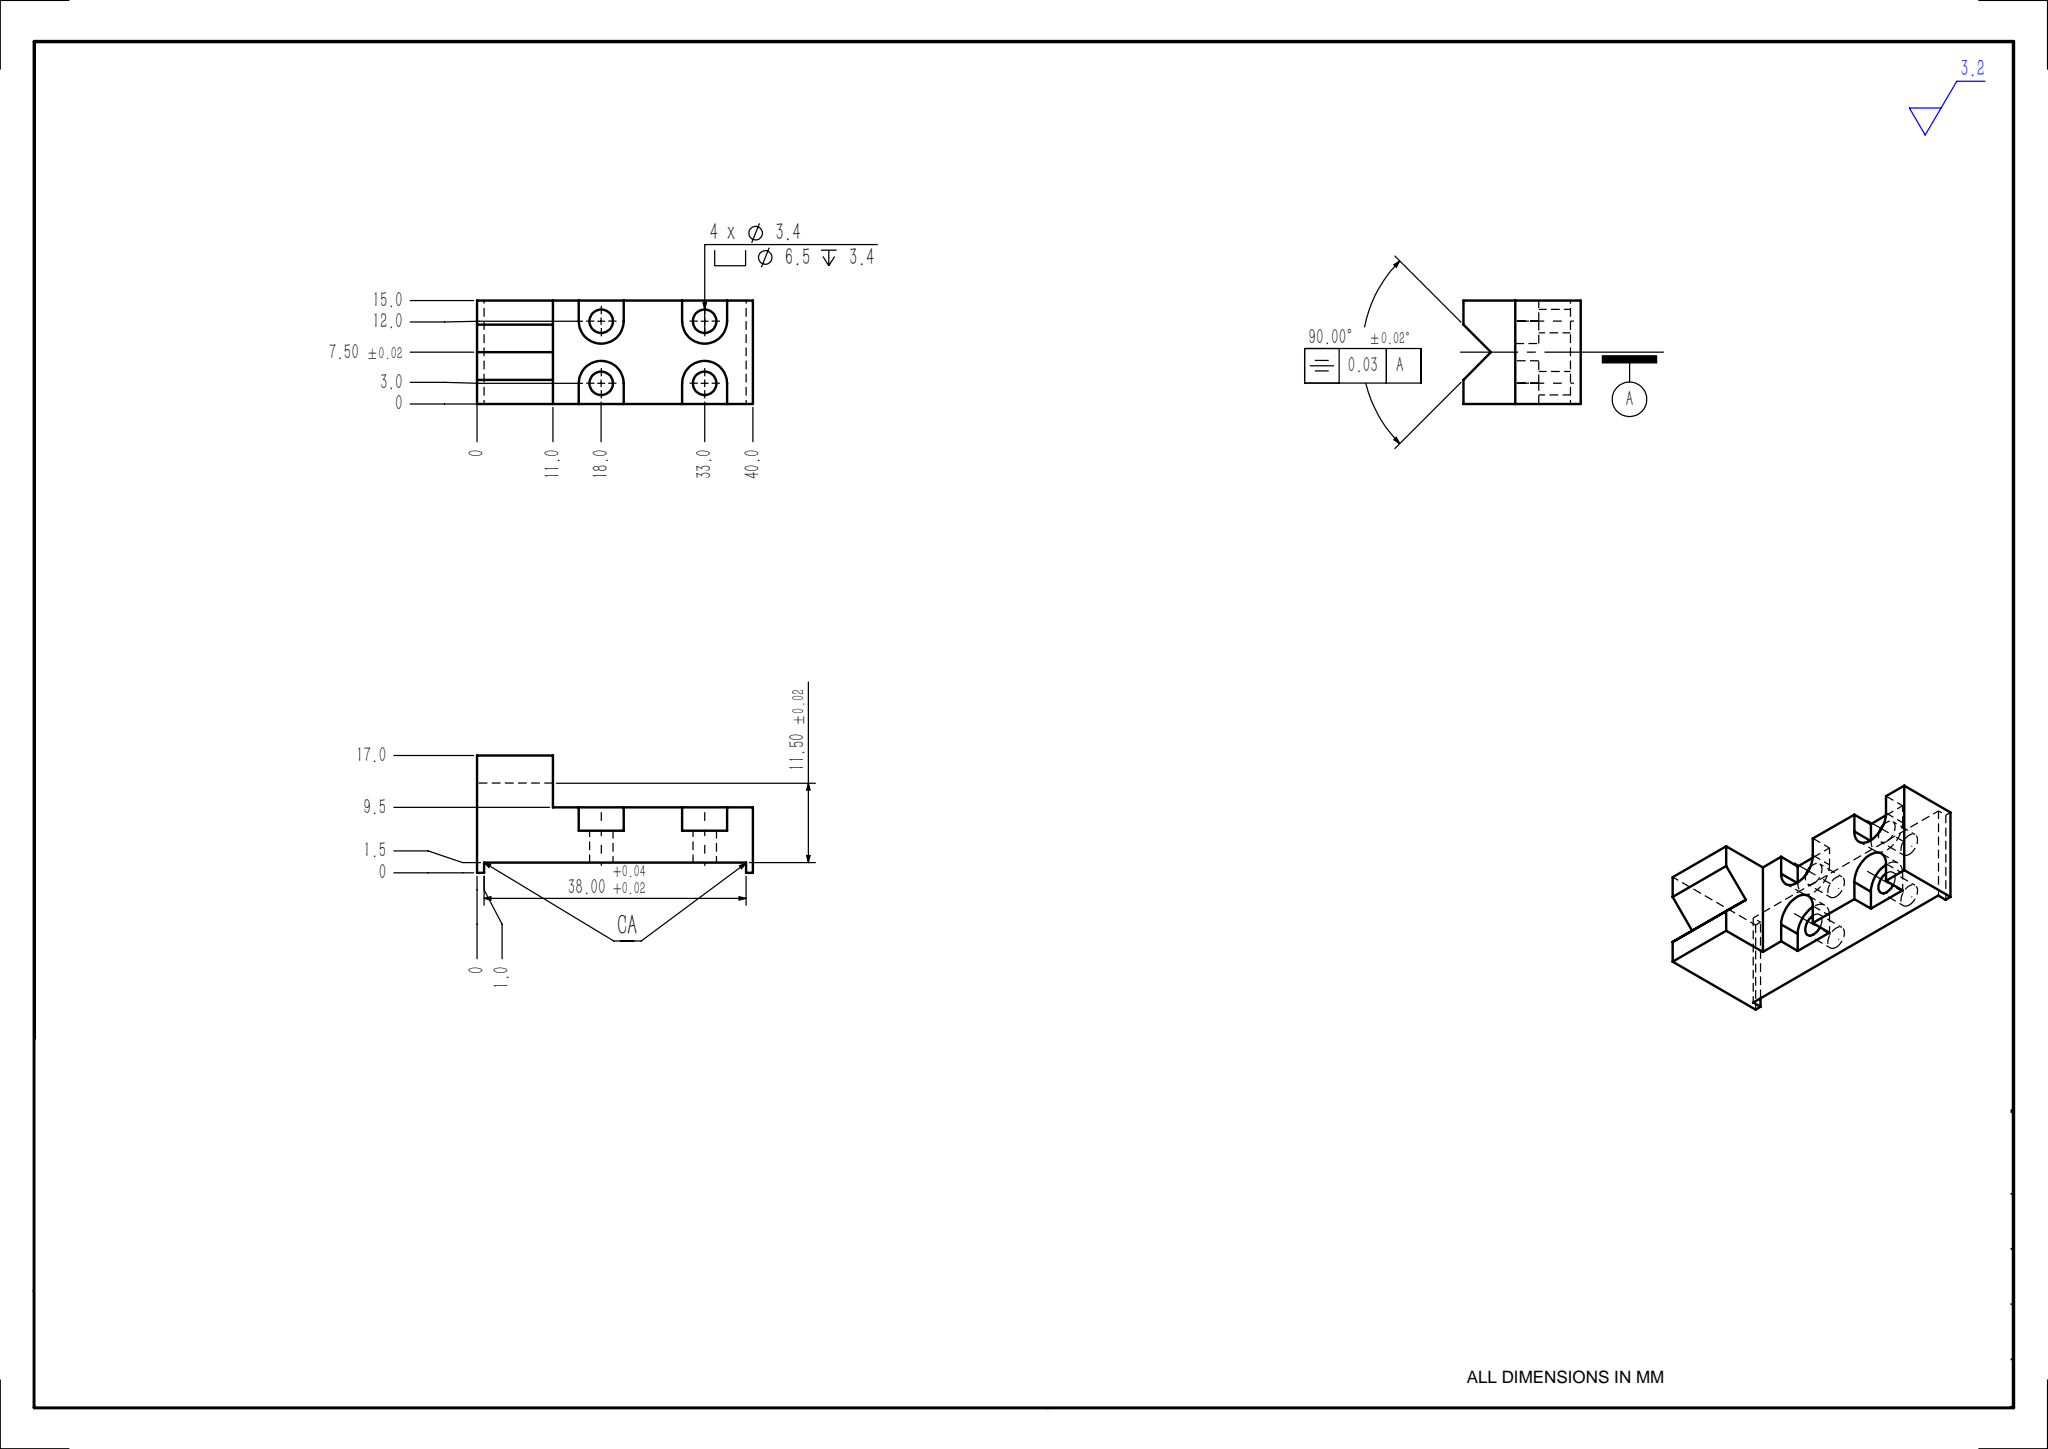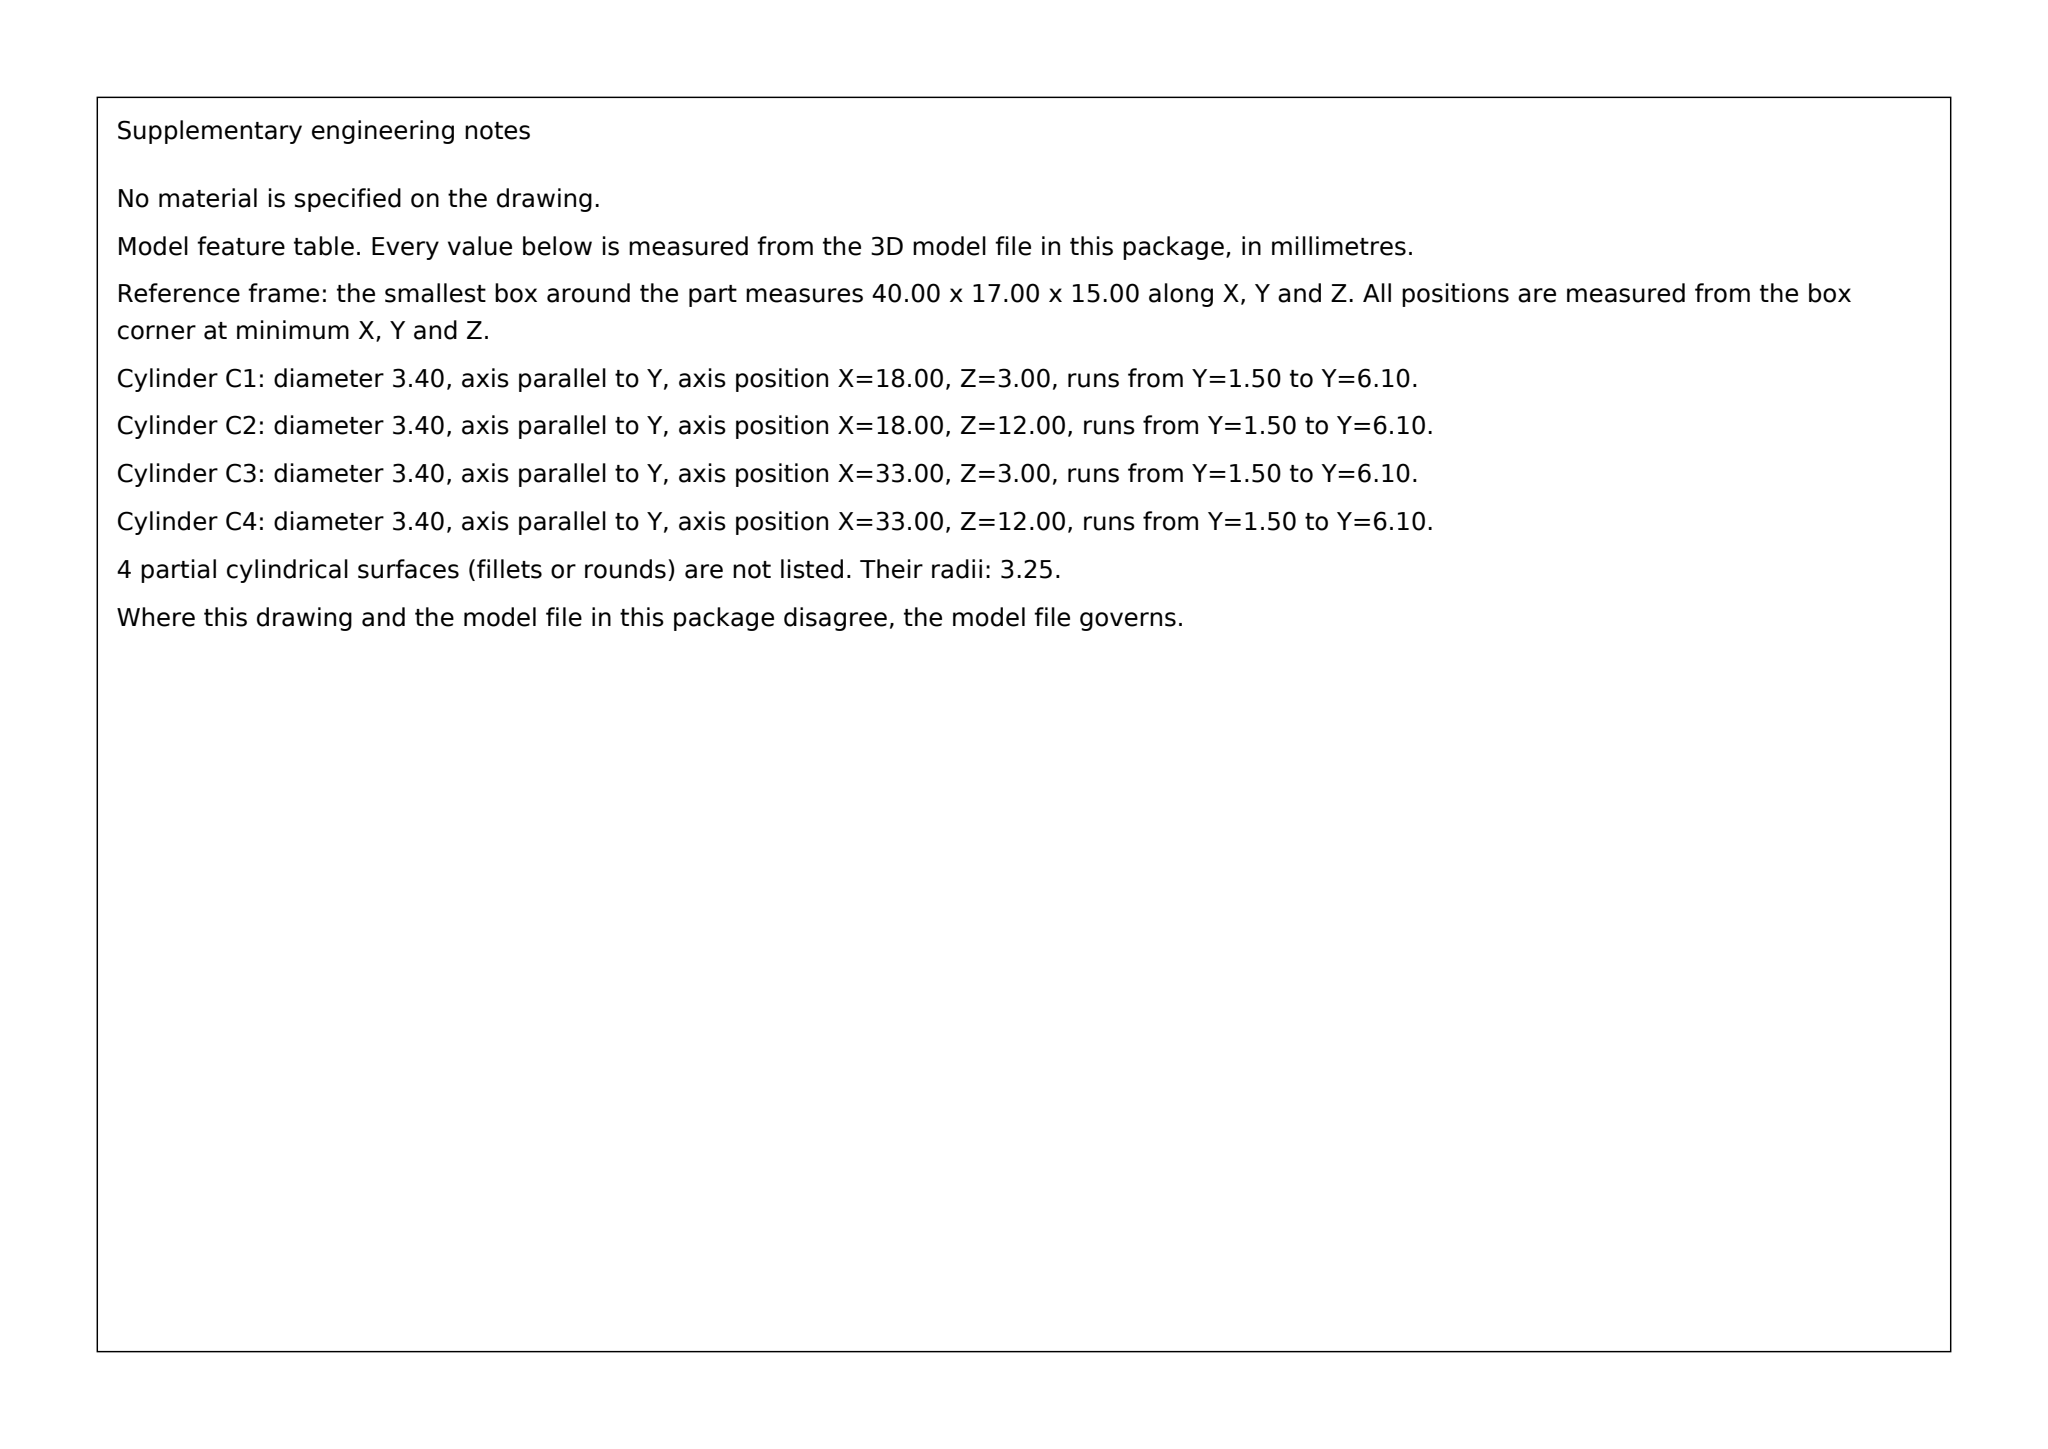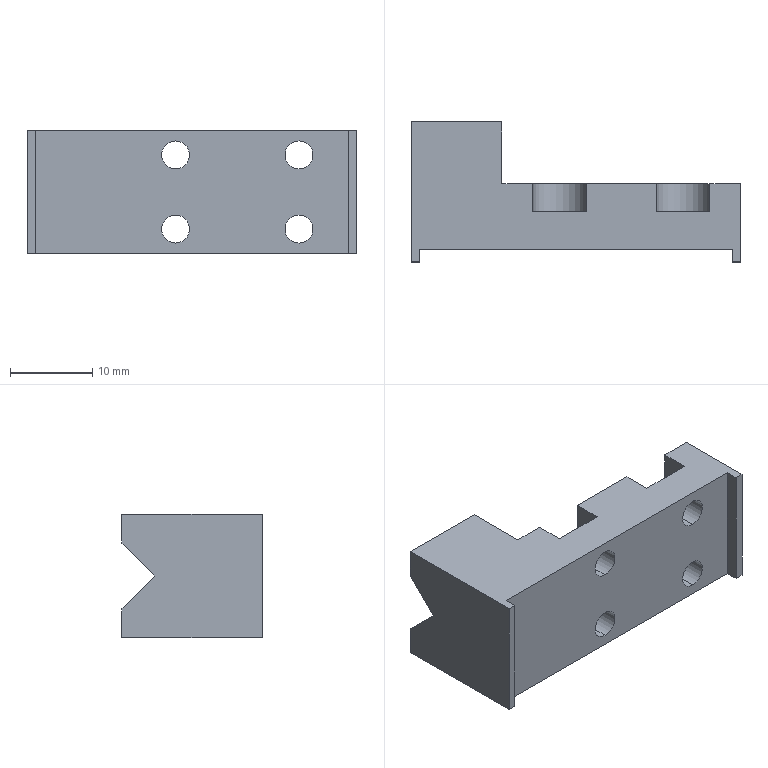Part | SolidWorks | mm | 1 solid | 41 faces | box 40 x 17 x 15 mm | volume 5249 mm3 | plane 27 | cylinder 14 | commonest cylinder face diameters 3.4 x8 6.5 x6
build123d program:
from build123d import *

# Parameters (mm, degrees)
BOSS_EXTRUDE1_DEPTH                             = 7.5
SKETCH2_W                                       = 29
SKETCH2_H                                       = 7.5
CUT_EXTRUDE1_DEPTH                              = 27.405
CUT_EXTRUDE2_DEPTH                              = 42.575
M3_HEX_SOCKET_HEAD_CAP_SCREW_CBORE1_D           = 3.4
M3_HEX_SOCKET_HEAD_CAP_SCREW_CBORE1_CBORE_D     = 6.5
M3_HEX_SOCKET_HEAD_CAP_SCREW_CBORE1_CBORE_DEPTH = 3.4
SKETCH6_W                                       = 6.5
SKETCH6_H                                       = 3
CUT_EXTRUDE3_DEPTH                              = 3.4


with BuildPart() as part:
    # Sketch1 → Boss-Extrude1 (new, symmetric)
    with BuildSketch(Plane.XY):
        Polygon((-19, -8.5), (-19, -7), (19, -7), (19, -8.5), (20, -8.5), (20, 8.5), (-20, 8.5), (-20, -8.5), align=None)
    extrude(amount=BOSS_EXTRUDE1_DEPTH, both=True)

    # Sketch2 → Cut-Extrude1 (cut, through all)
    with BuildSketch(Plane.XY.offset(7.5)):
        with Locations((5.5, 4.75)):
            Rectangle(SKETCH2_W, SKETCH2_H)
    extrude(amount=-CUT_EXTRUDE1_DEPTH, mode=Mode.SUBTRACT)

    # Sketch3 → Cut-Extrude2 (cut, through all)
    with BuildSketch(Plane.ZY.offset(20)):
        Polygon((-4, 8.5), (0, 4.5), (4, 8.5), align=None)
    extrude(amount=-CUT_EXTRUDE2_DEPTH, mode=Mode.SUBTRACT)

    # M3 Hex Socket Head Cap Screw CBORE1 (through all)
    with Locations(Plane(origin=(0, 1, 0), x_dir=(1, 0, 0), z_dir=(0, 1, 0))):
        with Locations((13, -4.5), (-2, -4.5), (13, 4.5), (-2, 4.5)):
            CounterBoreHole(M3_HEX_SOCKET_HEAD_CAP_SCREW_CBORE1_D / 2, M3_HEX_SOCKET_HEAD_CAP_SCREW_CBORE1_CBORE_D / 2, M3_HEX_SOCKET_HEAD_CAP_SCREW_CBORE1_CBORE_DEPTH)

    # Sketch6 → Cut-Extrude3 (cut)
    with BuildSketch(Plane(origin=(0, 1, 0), x_dir=(1, 0, 0), z_dir=(0, 1, 0))):
        with Locations((13, -6)):
            Rectangle(SKETCH6_W, SKETCH6_H)
        with Locations((-2, -6)):
            Rectangle(SKETCH6_W, SKETCH6_H)
        with Locations((13, 6)):
            Rectangle(SKETCH6_W, SKETCH6_H)
        with Locations((-2, 6)):
            Rectangle(SKETCH6_W, SKETCH6_H)
    extrude(amount=-CUT_EXTRUDE3_DEPTH, mode=Mode.SUBTRACT)


solid = part.part